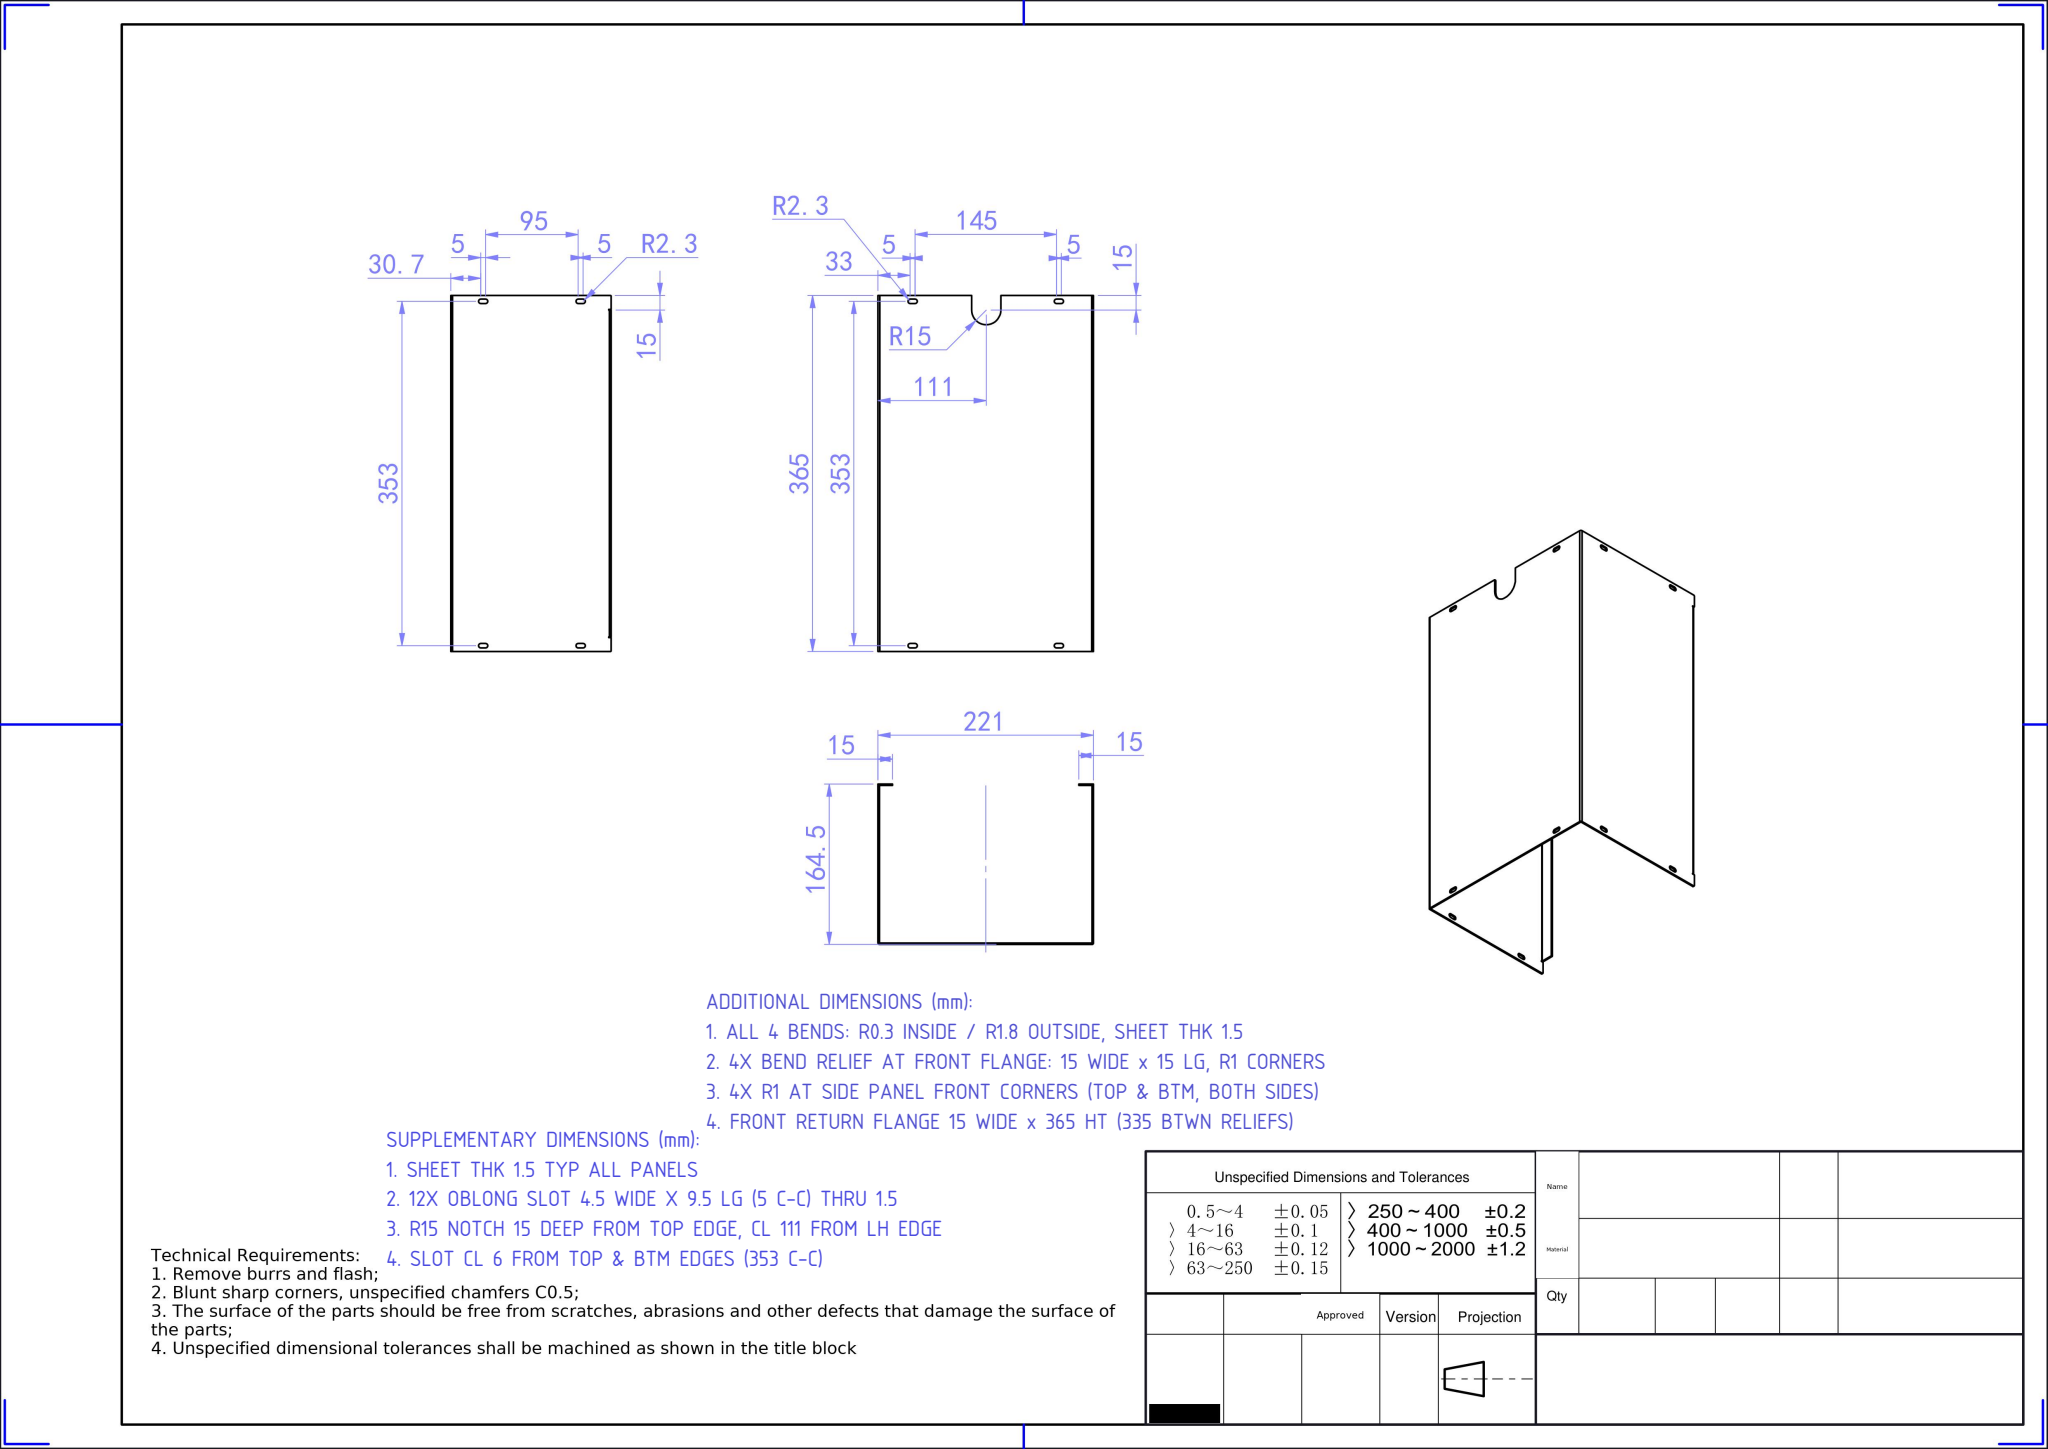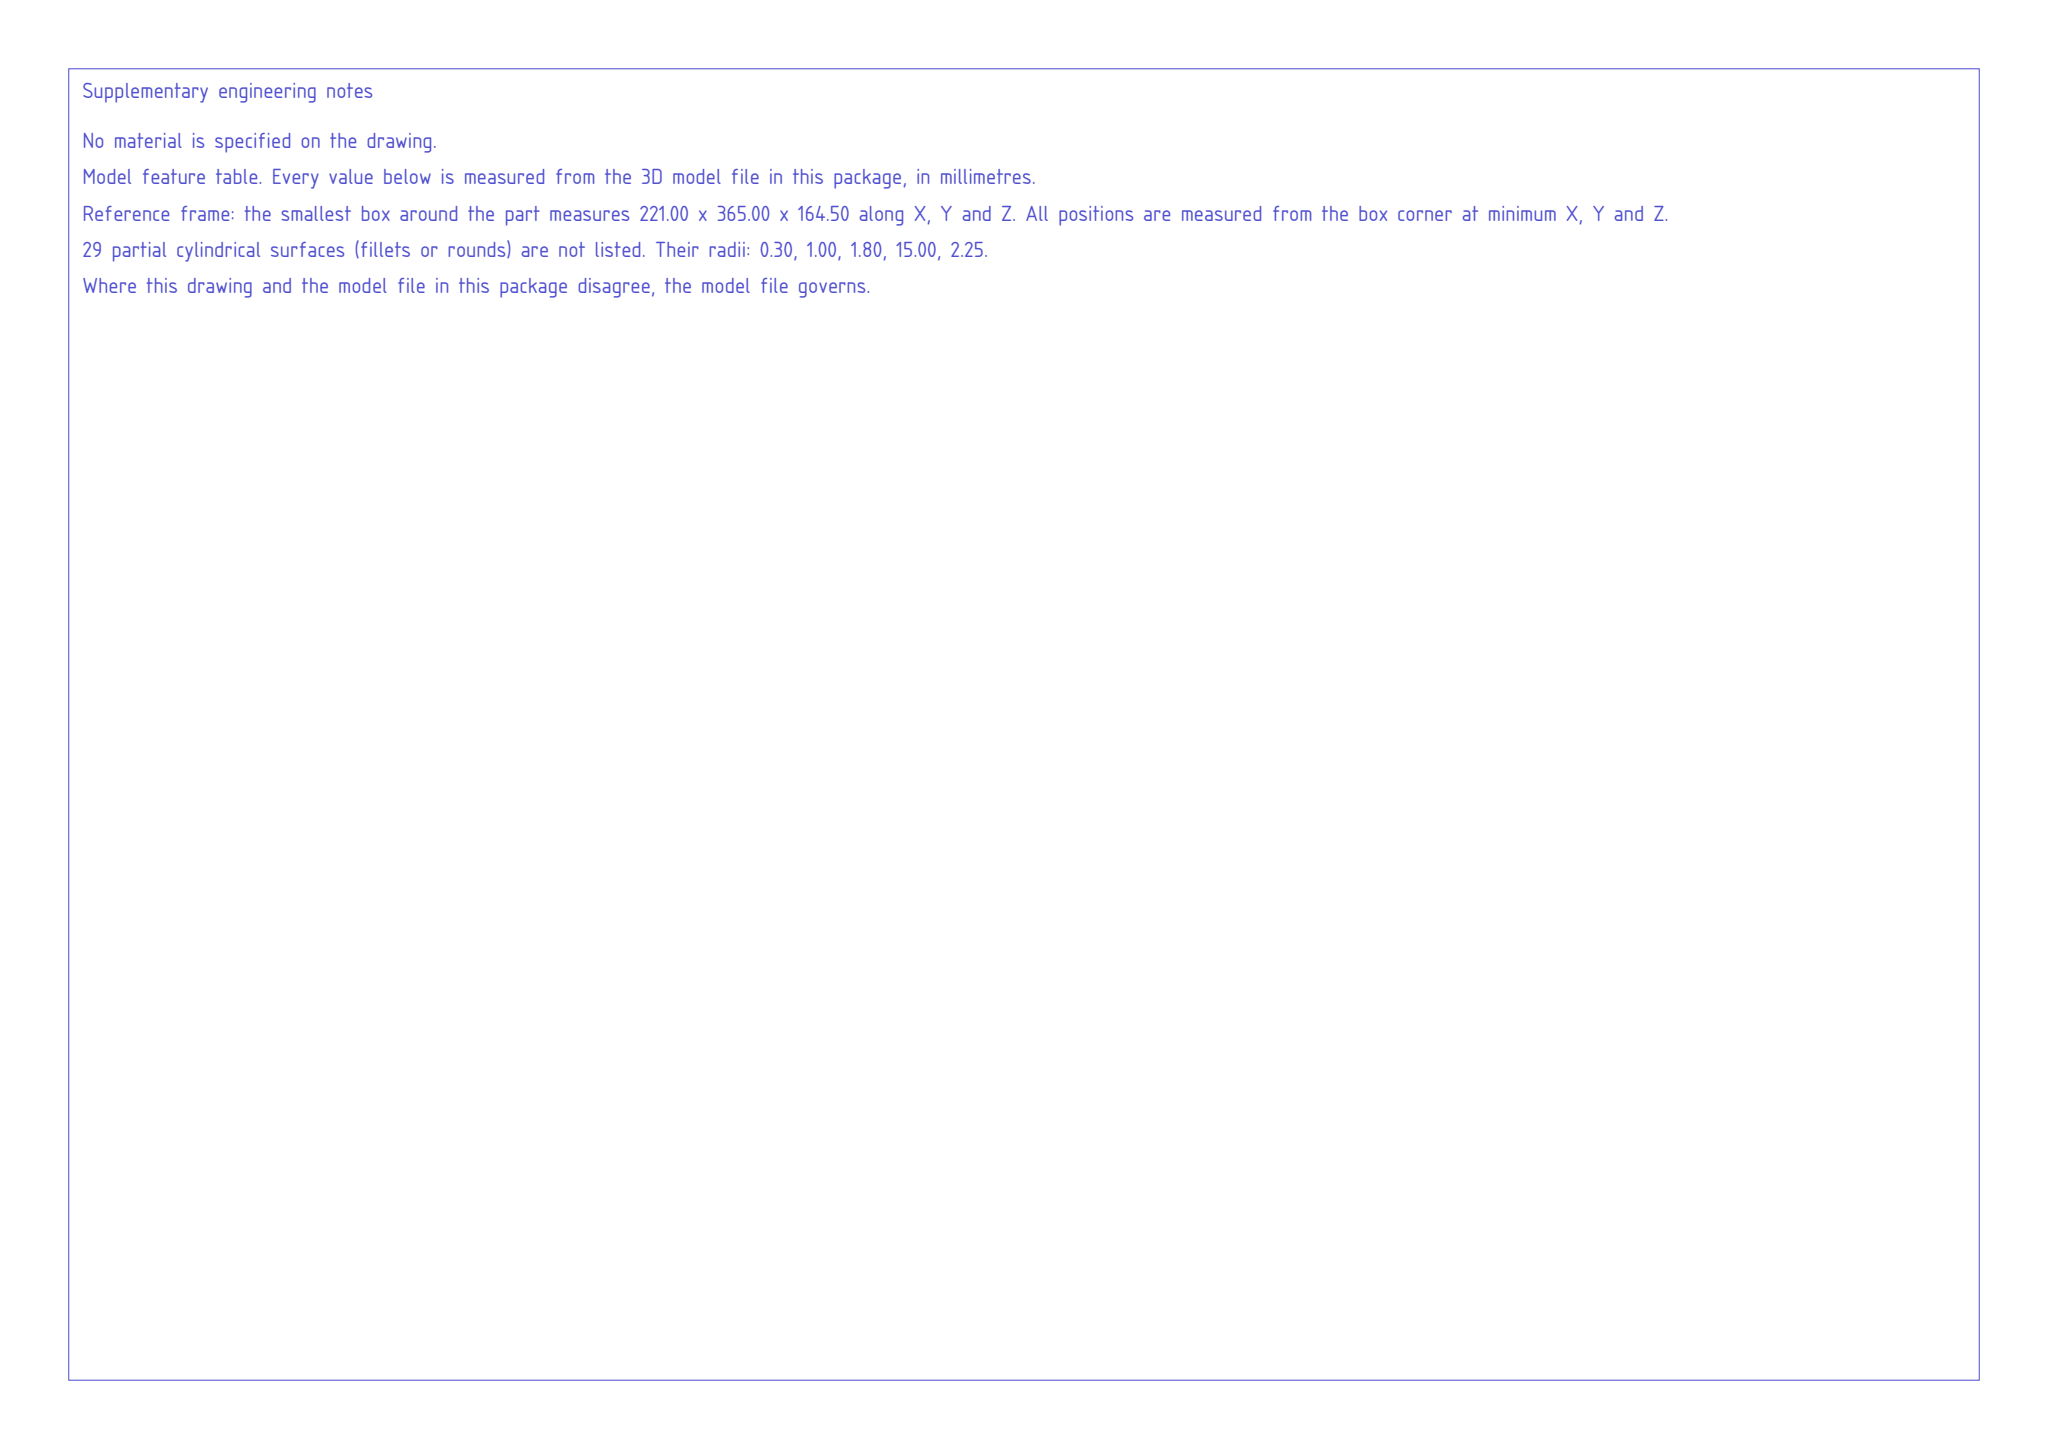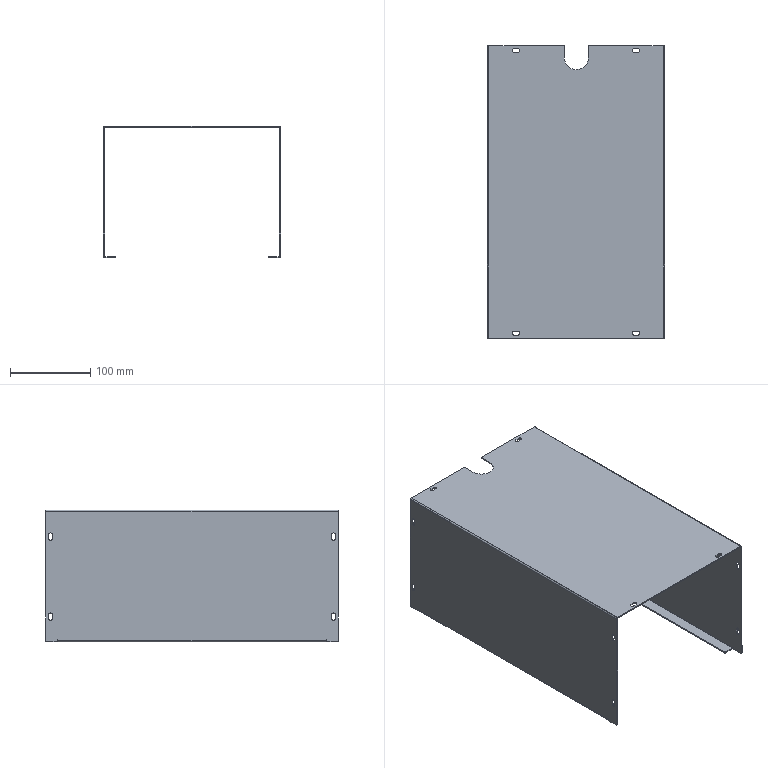Part | SolidWorks | mm | 1 solid | 124 faces | box 221 x 365 x 164.5 mm | volume 310194 mm3 | plane 73 | cylinder 51 | commonest cylinder face diameters 4.5 x36 2 x6 3.6 x4 0.6 x4 30 x1